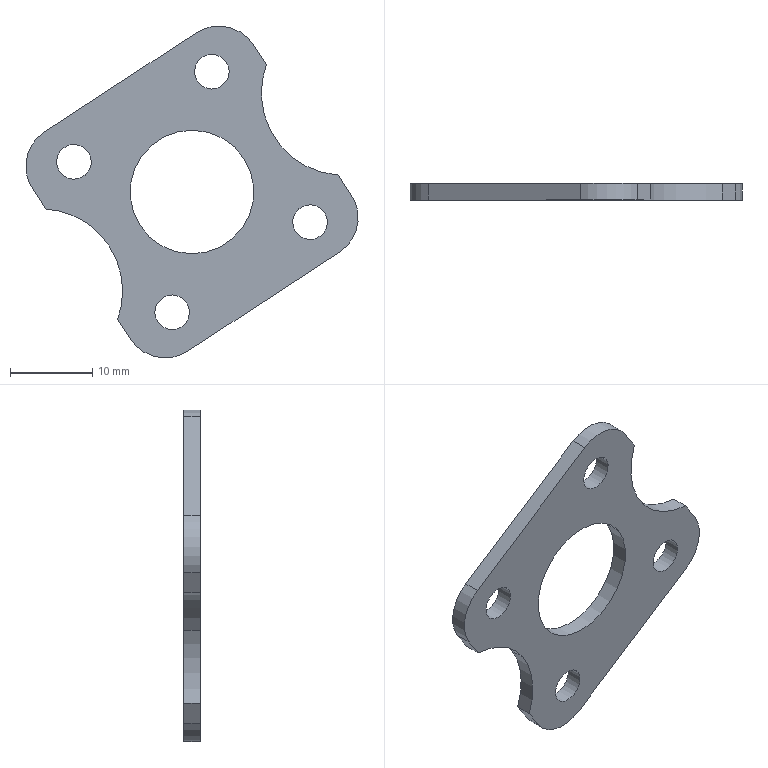Component | SolidWorks | FrontWheelPadPlate-2 | 1 solid | 25 faces | box 40.34 x 2 x 40.28 mm | volume 1349 mm3 | cylinder 17 | plane 8 | commonest cylinder face diameters 4.2 x8 10 x4 20 x3 15 x2
build123d program:
from build123d import *

# Parameters (mm, degrees)
SKETCH1_W           = 32
SKETCH1_H           = 31.8
SKETCH1_R           = 2.1
SKETCH1_R_2         = 7.5
BOSS_EXTRUDE1_DEPTH = 2
SKETCH2_R           = 10
CUT_EXTRUDE1_DEPTH  = 23.645
FILLET1_R           = 5


with BuildPart() as part:
    # Sketch1 → Boss-Extrude1 (new body)
    with BuildSketch(Plane.XY):
        Rectangle(SKETCH1_W, SKETCH1_H)
        with Locations((-10, 10.9)):
            Circle(SKETCH1_R, mode=Mode.SUBTRACT)
        with Locations(Location((10, 10.9, 0), (0, 0, 180))):
            Circle(SKETCH1_R, mode=Mode.SUBTRACT)
        with Locations((10, -10.9)):
            Circle(SKETCH1_R, mode=Mode.SUBTRACT)
        with Locations(Location((-10, -10.9, 0), (0, 0, 180))):
            Circle(SKETCH1_R, mode=Mode.SUBTRACT)
        Circle(SKETCH1_R_2, mode=Mode.SUBTRACT)
    extrude(amount=BOSS_EXTRUDE1_DEPTH)

    # Sketch2 → Cut-Extrude1 (cut, through all)
    with BuildSketch(Plane.XY.offset(2)):
        with Locations((22, 0)):
            Circle(SKETCH2_R)
        with Locations((-22, 0)):
            Circle(SKETCH2_R)
    extrude(amount=-CUT_EXTRUDE1_DEPTH, mode=Mode.SUBTRACT)

    # Fillet1
    fillet1_edges = [part.edges().sort_by_distance(p)[0] for p in [
        (16, -15.9, 1),
        (-16, -15.9, 1),
        (-16, 15.9, 1),
        (16, 15.9, 1),
    ]]
    fillet(fillet1_edges, radius=FILLET1_R)


solid = part.part

# Placed as in the assembly
solid = solid.moved(Location((0.3183, -13.6, 37), (90, 0, 33.158)))
STEP:
#1=CARTESIAN_POINT('',(-0.383,-0.6142,1.198));
#2=VERTEX_POINT('',#1);
#3=CARTESIAN_POINT('',(-0.3426,-0.6142,0.8485));
#4=VERTEX_POINT('',#3);
#5=CARTESIAN_POINT('',(-0.7126,-0.6142,0.983));
#6=DIRECTION('',(0.,1.,0.));
#7=DIRECTION('',(-0.8372,0.,-0.5469));
#8=AXIS2_PLACEMENT_3D('',#5,#6,#7);
#9=CIRCLE('',#8,0.3937);
#10=EDGE_CURVE('',#2,#4,#9,.T.);
#11=ORIENTED_EDGE('',*,*,#10,.F.);
#12=CARTESIAN_POINT('',(-0.383,-0.5354,1.198));
#13=VERTEX_POINT('',#12);
#14=CARTESIAN_POINT('',(-0.383,-0.6142,1.198));
#15=DIRECTION('',(0.,1.,0.));
#16=VECTOR('',#15,39.37);
#17=LINE('',#14,#16);
#18=EDGE_CURVE('',#2,#13,#17,.T.);
#19=ORIENTED_EDGE('',*,*,#18,.T.);
#20=CARTESIAN_POINT('',(-0.3426,-0.5354,0.8485));
#21=VERTEX_POINT('',#20);
#22=CARTESIAN_POINT('',(-0.7126,-0.5354,0.983));
#23=DIRECTION('',(0.,1.,0.));
#24=DIRECTION('',(-0.8372,0.,-0.5469));
#25=AXIS2_PLACEMENT_3D('',#22,#23,#24);
#26=CIRCLE('',#25,0.3937);
#27=EDGE_CURVE('',#13,#21,#26,.T.);
#28=ORIENTED_EDGE('',*,*,#27,.T.);
#29=CARTESIAN_POINT('',(-0.3426,-0.6142,0.8485));
#30=DIRECTION('',(0.,1.,0.));
#31=VECTOR('',#30,39.37);
#32=LINE('',#29,#31);
#33=EDGE_CURVE('',#4,#21,#32,.T.);
#34=ORIENTED_EDGE('',*,*,#33,.F.);
#35=EDGE_LOOP('',(#11,#19,#28,#34));
#36=FACE_OUTER_BOUND('',#35,.T.);
#37=CARTESIAN_POINT('',(-0.7126,-0.6142,0.983));
#38=DIRECTION('',(0.,1.,0.));
#39=DIRECTION('',(0.8372,0.,0.5469));
#40=AXIS2_PLACEMENT_3D('',#37,#38,#39);
#41=CYLINDRICAL_SURFACE('',#40,0.3937);
#42=ADVANCED_FACE('',(#36),#41,.F.);
#43=CARTESIAN_POINT('',(-0.2347,-0.5354,1.295));
#44=VERTEX_POINT('',#43);
#45=CARTESIAN_POINT('',(0.2597,-0.5354,1.618));
#46=VERTEX_POINT('',#45);
#47=CARTESIAN_POINT('',(0.01253,-0.5354,1.457));
#48=DIRECTION('',(0.,1.,0.));
#49=DIRECTION('',(0.8372,0.,0.5469));
#50=AXIS2_PLACEMENT_3D('',#47,#48,#49);
#51=CIRCLE('',#50,0.2953);
#52=EDGE_CURVE('',#44,#46,#51,.T.);
#53=ORIENTED_EDGE('',*,*,#52,.T.);
#54=CARTESIAN_POINT('',(0.2597,-0.6142,1.618));
#55=VERTEX_POINT('',#54);
#56=CARTESIAN_POINT('',(0.2597,-0.5354,1.618));
#57=DIRECTION('',(0.,-1.,0.));
#58=VECTOR('',#57,39.37);
#59=LINE('',#56,#58);
#60=EDGE_CURVE('',#46,#55,#59,.T.);
#61=ORIENTED_EDGE('',*,*,#60,.T.);
#62=CARTESIAN_POINT('',(-0.2347,-0.6142,1.295));
#63=VERTEX_POINT('',#62);
#64=CARTESIAN_POINT('',(0.01253,-0.6142,1.457));
#65=DIRECTION('',(0.,1.,0.));
#66=DIRECTION('',(0.8372,0.,0.5469));
#67=AXIS2_PLACEMENT_3D('',#64,#65,#66);
#68=CIRCLE('',#67,0.2953);
#69=EDGE_CURVE('',#63,#55,#68,.T.);
#70=ORIENTED_EDGE('',*,*,#69,.F.);
#71=CARTESIAN_POINT('',(-0.2347,-0.5354,1.295));
#72=DIRECTION('',(0.,-1.,0.));
#73=VECTOR('',#72,39.37);
#74=LINE('',#71,#73);
#75=EDGE_CURVE('',#44,#63,#74,.T.);
#76=ORIENTED_EDGE('',*,*,#75,.F.);
#77=EDGE_LOOP('',(#53,#61,#70,#76));
#78=FACE_OUTER_BOUND('',#77,.T.);
#79=CARTESIAN_POINT('',(0.01253,-0.5354,1.457));
#80=DIRECTION('',(0.,-1.,0.));
#81=DIRECTION('',(-0.8372,0.,-0.5469));
#82=AXIS2_PLACEMENT_3D('',#79,#80,#81);
#83=CYLINDRICAL_SURFACE('',#82,0.2953);
#84=ADVANCED_FACE('',(#78),#83,.F.);
#85=CARTESIAN_POINT('',(-0.621,-0.5354,1.555));
#86=VERTEX_POINT('',#85);
#87=CARTESIAN_POINT('',(-0.4826,-0.5354,1.646));
#88=VERTEX_POINT('',#87);
#89=CARTESIAN_POINT('',(-0.5518,-0.5354,1.601));
#90=DIRECTION('',(0.,1.,0.));
#91=DIRECTION('',(-0.8372,0.,-0.5469));
#92=AXIS2_PLACEMENT_3D('',#89,#90,#91);
#93=CIRCLE('',#92,0.08268);
#94=EDGE_CURVE('',#86,#88,#93,.T.);
#95=ORIENTED_EDGE('',*,*,#94,.T.);
#96=CARTESIAN_POINT('',(-0.4826,-0.6142,1.646));
#97=VERTEX_POINT('',#96);
#98=CARTESIAN_POINT('',(-0.4826,-0.5354,1.646));
#99=DIRECTION('',(0.,-1.,0.));
#100=VECTOR('',#99,39.37);
#101=LINE('',#98,#100);
#102=EDGE_CURVE('',#88,#97,#101,.T.);
#103=ORIENTED_EDGE('',*,*,#102,.T.);
#104=CARTESIAN_POINT('',(-0.621,-0.6142,1.555));
#105=VERTEX_POINT('',#104);
#106=CARTESIAN_POINT('',(-0.5518,-0.6142,1.601));
#107=DIRECTION('',(0.,1.,0.));
#108=DIRECTION('',(-0.8372,0.,-0.5469));
#109=AXIS2_PLACEMENT_3D('',#106,#107,#108);
#110=CIRCLE('',#109,0.08268);
#111=EDGE_CURVE('',#105,#97,#110,.T.);
#112=ORIENTED_EDGE('',*,*,#111,.F.);
#113=CARTESIAN_POINT('',(-0.621,-0.5354,1.555));
#114=DIRECTION('',(0.,-1.,0.));
#115=VECTOR('',#114,39.37);
#116=LINE('',#113,#115);
#117=EDGE_CURVE('',#86,#105,#116,.T.);
#118=ORIENTED_EDGE('',*,*,#117,.F.);
#119=EDGE_LOOP('',(#95,#103,#112,#118));
#120=FACE_OUTER_BOUND('',#119,.T.);
#121=CARTESIAN_POINT('',(-0.5518,-0.5354,1.601));
#122=DIRECTION('',(0.,-1.,0.));
#123=DIRECTION('',(-0.8372,0.,-0.5469));
#124=AXIS2_PLACEMENT_3D('',#121,#122,#123);
#125=CYLINDRICAL_SURFACE('',#124,0.08268);
#126=ADVANCED_FACE('',(#120),#125,.F.);
#127=CARTESIAN_POINT('',(0.0382,-0.5354,1.986));
#128=VERTEX_POINT('',#127);
#129=CARTESIAN_POINT('',(0.1766,-0.5354,2.077));
#130=VERTEX_POINT('',#129);
#131=CARTESIAN_POINT('',(0.1074,-0.5354,2.031));
#132=DIRECTION('',(0.,1.,0.));
#133=DIRECTION('',(0.8372,0.,0.5469));
#134=AXIS2_PLACEMENT_3D('',#131,#132,#133);
#135=CIRCLE('',#134,0.08268);
#136=EDGE_CURVE('',#128,#130,#135,.T.);
#137=ORIENTED_EDGE('',*,*,#136,.T.);
#138=CARTESIAN_POINT('',(0.1766,-0.6142,2.077));
#139=VERTEX_POINT('',#138);
#140=CARTESIAN_POINT('',(0.1766,-0.5354,2.077));
#141=DIRECTION('',(0.,-1.,0.));
#142=VECTOR('',#141,39.37);
#143=LINE('',#140,#142);
#144=EDGE_CURVE('',#130,#139,#143,.T.);
#145=ORIENTED_EDGE('',*,*,#144,.T.);
#146=CARTESIAN_POINT('',(0.0382,-0.6142,1.986));
#147=VERTEX_POINT('',#146);
#148=CARTESIAN_POINT('',(0.1074,-0.6142,2.031));
#149=DIRECTION('',(0.,1.,0.));
#150=DIRECTION('',(0.8372,0.,0.5469));
#151=AXIS2_PLACEMENT_3D('',#148,#149,#150);
#152=CIRCLE('',#151,0.08268);
#153=EDGE_CURVE('',#147,#139,#152,.T.);
#154=ORIENTED_EDGE('',*,*,#153,.F.);
#155=CARTESIAN_POINT('',(0.0382,-0.5354,1.986));
#156=DIRECTION('',(0.,-1.,0.));
#157=VECTOR('',#156,39.37);
#158=LINE('',#155,#157);
#159=EDGE_CURVE('',#128,#147,#158,.T.);
#160=ORIENTED_EDGE('',*,*,#159,.F.);
#161=EDGE_LOOP('',(#137,#145,#154,#160));
#162=FACE_OUTER_BOUND('',#161,.T.);
#163=CARTESIAN_POINT('',(0.1074,-0.5354,2.031));
#164=DIRECTION('',(0.,-1.,0.));
#165=DIRECTION('',(-0.8372,0.,-0.5469));
#166=AXIS2_PLACEMENT_3D('',#163,#164,#165);
#167=CYLINDRICAL_SURFACE('',#166,0.08268);
#168=ADVANCED_FACE('',(#162),#167,.F.);
#169=CARTESIAN_POINT('',(0.5076,-0.5354,1.268));
#170=VERTEX_POINT('',#169);
#171=CARTESIAN_POINT('',(0.6461,-0.5354,1.358));
#172=VERTEX_POINT('',#171);
#173=CARTESIAN_POINT('',(0.5768,-0.5354,1.313));
#174=DIRECTION('',(0.,1.,0.));
#175=DIRECTION('',(-0.8372,0.,-0.5469));
#176=AXIS2_PLACEMENT_3D('',#173,#174,#175);
#177=CIRCLE('',#176,0.08268);
#178=EDGE_CURVE('',#170,#172,#177,.T.);
#179=ORIENTED_EDGE('',*,*,#178,.T.);
#180=CARTESIAN_POINT('',(0.6461,-0.6142,1.358));
#181=VERTEX_POINT('',#180);
#182=CARTESIAN_POINT('',(0.6461,-0.5354,1.358));
#183=DIRECTION('',(0.,-1.,0.));
#184=VECTOR('',#183,39.37);
#185=LINE('',#182,#184);
#186=EDGE_CURVE('',#172,#181,#185,.T.);
#187=ORIENTED_EDGE('',*,*,#186,.T.);
#188=CARTESIAN_POINT('',(0.5076,-0.6142,1.268));
#189=VERTEX_POINT('',#188);
#190=CARTESIAN_POINT('',(0.5768,-0.6142,1.313));
#191=DIRECTION('',(0.,1.,0.));
#192=DIRECTION('',(-0.8372,0.,-0.5469));
#193=AXIS2_PLACEMENT_3D('',#190,#191,#192);
#194=CIRCLE('',#193,0.08268);
#195=EDGE_CURVE('',#189,#181,#194,.T.);
#196=ORIENTED_EDGE('',*,*,#195,.F.);
#197=CARTESIAN_POINT('',(0.5076,-0.5354,1.268));
#198=DIRECTION('',(0.,-1.,0.));
#199=VECTOR('',#198,39.37);
#200=LINE('',#197,#199);
#201=EDGE_CURVE('',#170,#189,#200,.T.);
#202=ORIENTED_EDGE('',*,*,#201,.F.);
#203=EDGE_LOOP('',(#179,#187,#196,#202));
#204=FACE_OUTER_BOUND('',#203,.T.);
#205=CARTESIAN_POINT('',(0.5768,-0.5354,1.313));
#206=DIRECTION('',(0.,-1.,0.));
#207=DIRECTION('',(-0.8372,0.,-0.5469));
#208=AXIS2_PLACEMENT_3D('',#205,#206,#207);
#209=CYLINDRICAL_SURFACE('',#208,0.08268);
#210=ADVANCED_FACE('',(#204),#209,.F.);
#211=CARTESIAN_POINT('',(-0.1516,-0.5354,0.8369));
#212=VERTEX_POINT('',#211);
#213=CARTESIAN_POINT('',(-0.01313,-0.5354,0.9273));
#214=VERTEX_POINT('',#213);
#215=CARTESIAN_POINT('',(-0.08235,-0.5354,0.8821));
#216=DIRECTION('',(0.,1.,0.));
#217=DIRECTION('',(0.8372,0.,0.5469));
#218=AXIS2_PLACEMENT_3D('',#215,#216,#217);
#219=CIRCLE('',#218,0.08268);
#220=EDGE_CURVE('',#212,#214,#219,.T.);
#221=ORIENTED_EDGE('',*,*,#220,.T.);
#222=CARTESIAN_POINT('',(-0.01313,-0.6142,0.9273));
#223=VERTEX_POINT('',#222);
#224=CARTESIAN_POINT('',(-0.01313,-0.5354,0.9273));
#225=DIRECTION('',(0.,-1.,0.));
#226=VECTOR('',#225,39.37);
#227=LINE('',#224,#226);
#228=EDGE_CURVE('',#214,#223,#227,.T.);
#229=ORIENTED_EDGE('',*,*,#228,.T.);
#230=CARTESIAN_POINT('',(-0.1516,-0.6142,0.8369));
#231=VERTEX_POINT('',#230);
#232=CARTESIAN_POINT('',(-0.08235,-0.6142,0.8821));
#233=DIRECTION('',(0.,1.,0.));
#234=DIRECTION('',(0.8372,0.,0.5469));
#235=AXIS2_PLACEMENT_3D('',#232,#233,#234);
#236=CIRCLE('',#235,0.08268);
#237=EDGE_CURVE('',#231,#223,#236,.T.);
#238=ORIENTED_EDGE('',*,*,#237,.F.);
#239=CARTESIAN_POINT('',(-0.1516,-0.5354,0.8369));
#240=DIRECTION('',(0.,-1.,0.));
#241=VECTOR('',#240,39.37);
#242=LINE('',#239,#241);
#243=EDGE_CURVE('',#212,#231,#242,.T.);
#244=ORIENTED_EDGE('',*,*,#243,.F.);
#245=EDGE_LOOP('',(#221,#229,#238,#244));
#246=FACE_OUTER_BOUND('',#245,.T.);
#247=CARTESIAN_POINT('',(-0.08235,-0.5354,0.8821));
#248=DIRECTION('',(0.,-1.,0.));
#249=DIRECTION('',(-0.8372,0.,-0.5469));
#250=AXIS2_PLACEMENT_3D('',#247,#248,#249);
#251=CYLINDRICAL_SURFACE('',#250,0.08268);
#252=ADVANCED_FACE('',(#246),#251,.F.);
#253=CARTESIAN_POINT('',(-0.2801,-0.5354,0.7529));
#254=VERTEX_POINT('',#253);
#255=CARTESIAN_POINT('',(-0.8572,-0.5354,1.636));
#256=DIRECTION('',(-0.5469,0.,0.8372));
#257=VECTOR('',#256,39.37);
#258=LINE('',#255,#257);
#259=EDGE_CURVE('',#254,#21,#258,.T.);
#260=ORIENTED_EDGE('',*,*,#259,.F.);
#261=CARTESIAN_POINT('',(-0.2801,-0.6142,0.7529));
#262=VERTEX_POINT('',#261);
#263=CARTESIAN_POINT('',(-0.2801,-0.5354,0.7529));
#264=DIRECTION('',(0.,-1.,0.));
#265=VECTOR('',#264,39.37);
#266=LINE('',#263,#265);
#267=EDGE_CURVE('',#254,#262,#266,.T.);
#268=ORIENTED_EDGE('',*,*,#267,.T.);
#269=CARTESIAN_POINT('',(-0.8572,-0.6142,1.636));
#270=DIRECTION('',(-0.5469,0.,0.8372));
#271=VECTOR('',#270,39.37);
#272=LINE('',#269,#271);
#273=EDGE_CURVE('',#262,#4,#272,.T.);
#274=ORIENTED_EDGE('',*,*,#273,.T.);
#275=ORIENTED_EDGE('',*,*,#33,.T.);
#276=EDGE_LOOP('',(#260,#268,#274,#275));
#277=FACE_OUTER_BOUND('',#276,.T.);
#278=CARTESIAN_POINT('',(-0.8572,-0.5354,1.636));
#279=DIRECTION('',(0.8372,0.,0.5469));
#280=DIRECTION('',(0.,-1.,0.));
#281=AXIS2_PLACEMENT_3D('',#278,#279,#280);
#282=PLANE('',#281);
#283=ADVANCED_FACE('',(#277),#282,.F.);
#284=CARTESIAN_POINT('',(0.3052,-0.5354,2.16));
#285=VERTEX_POINT('',#284);
#286=CARTESIAN_POINT('',(0.3676,-0.5354,2.065));
#287=VERTEX_POINT('',#286);
#288=CARTESIAN_POINT('',(0.1975,-0.5354,2.325));
#289=DIRECTION('',(0.5469,0.,-0.8372));
#290=VECTOR('',#289,39.37);
#291=LINE('',#288,#290);
#292=EDGE_CURVE('',#285,#287,#291,.T.);
#293=ORIENTED_EDGE('',*,*,#292,.F.);
#294=CARTESIAN_POINT('',(0.3052,-0.6142,2.16));
#295=VERTEX_POINT('',#294);
#296=CARTESIAN_POINT('',(0.3052,-0.5354,2.16));
#297=DIRECTION('',(0.,-1.,0.));
#298=VECTOR('',#297,39.37);
#299=LINE('',#296,#298);
#300=EDGE_CURVE('',#285,#295,#299,.T.);
#301=ORIENTED_EDGE('',*,*,#300,.T.);
#302=CARTESIAN_POINT('',(0.3676,-0.6142,2.065));
#303=VERTEX_POINT('',#302);
#304=CARTESIAN_POINT('',(0.1975,-0.6142,2.325));
#305=DIRECTION('',(0.5469,0.,-0.8372));
#306=VECTOR('',#305,39.37);
#307=LINE('',#304,#306);
#308=EDGE_CURVE('',#295,#303,#307,.T.);
#309=ORIENTED_EDGE('',*,*,#308,.T.);
#310=CARTESIAN_POINT('',(0.3676,-0.6142,2.065));
#311=DIRECTION('',(0.,1.,0.));
#312=VECTOR('',#311,39.37);
#313=LINE('',#310,#312);
#314=EDGE_CURVE('',#303,#287,#313,.T.);
#315=ORIENTED_EDGE('',*,*,#314,.T.);
#316=EDGE_LOOP('',(#293,#301,#309,#315));
#317=FACE_OUTER_BOUND('',#316,.T.);
#318=CARTESIAN_POINT('',(0.1975,-0.5354,2.325));
#319=DIRECTION('',(-0.8372,0.,-0.5469));
#320=DIRECTION('',(0.,1.,0.));
#321=AXIS2_PLACEMENT_3D('',#318,#319,#320);
#322=PLANE('',#321);
#323=ADVANCED_FACE('',(#317),#322,.F.);
#324=CARTESIAN_POINT('',(-0.6871,-0.5354,1.376));
#325=VERTEX_POINT('',#324);
#326=CARTESIAN_POINT('',(-0.7495,-0.5354,1.471));
#327=VERTEX_POINT('',#326);
#328=CARTESIAN_POINT('',(-0.8572,-0.5354,1.636));
#329=DIRECTION('',(-0.5469,0.,0.8372));
#330=VECTOR('',#329,39.37);
#331=LINE('',#328,#330);
#332=EDGE_CURVE('',#325,#327,#331,.T.);
#333=ORIENTED_EDGE('',*,*,#332,.T.);
#334=CARTESIAN_POINT('',(-0.6924,-0.5354,1.744));
#335=VERTEX_POINT('',#334);
#336=CARTESIAN_POINT('',(-0.5847,-0.5354,1.579));
#337=DIRECTION('',(0.,1.,0.));
#338=DIRECTION('',(-0.8372,0.,-0.5469));
#339=AXIS2_PLACEMENT_3D('',#336,#337,#338);
#340=CIRCLE('',#339,0.1969);
#341=EDGE_CURVE('',#327,#335,#340,.T.);
#342=ORIENTED_EDGE('',*,*,#341,.T.);
#343=CARTESIAN_POINT('',(0.03271,-0.5354,2.218));
#344=VERTEX_POINT('',#343);
#345=CARTESIAN_POINT('',(-0.8572,-0.5354,1.636));
#346=DIRECTION('',(0.8372,0.,0.5469));
#347=VECTOR('',#346,39.37);
#348=LINE('',#345,#347);
#349=EDGE_CURVE('',#335,#344,#348,.T.);
#350=ORIENTED_EDGE('',*,*,#349,.T.);
#351=CARTESIAN_POINT('',(0.1404,-0.5354,2.053));
#352=DIRECTION('',(0.,1.,0.));
#353=DIRECTION('',(-0.8372,0.,-0.5469));
#354=AXIS2_PLACEMENT_3D('',#351,#352,#353);
#355=CIRCLE('',#354,0.1969);
#356=EDGE_CURVE('',#344,#285,#355,.T.);
#357=ORIENTED_EDGE('',*,*,#356,.T.);
#358=ORIENTED_EDGE('',*,*,#292,.T.);
#359=CARTESIAN_POINT('',(0.7121,-0.5354,1.538));
#360=VERTEX_POINT('',#359);
#361=CARTESIAN_POINT('',(0.7376,-0.5354,1.93));
#362=DIRECTION('',(0.,1.,0.));
#363=DIRECTION('',(0.8372,0.,0.5469));
#364=AXIS2_PLACEMENT_3D('',#361,#362,#363);
#365=CIRCLE('',#364,0.3937);
#366=EDGE_CURVE('',#360,#287,#365,.T.);
#367=ORIENTED_EDGE('',*,*,#366,.F.);
#368=CARTESIAN_POINT('',(0.7746,-0.5354,1.442));
#369=VERTEX_POINT('',#368);
#370=CARTESIAN_POINT('',(0.1975,-0.5354,2.325));
#371=DIRECTION('',(0.5469,0.,-0.8372));
#372=VECTOR('',#371,39.37);
#373=LINE('',#370,#372);
#374=EDGE_CURVE('',#360,#369,#373,.T.);
#375=ORIENTED_EDGE('',*,*,#374,.T.);
#376=CARTESIAN_POINT('',(0.7175,-0.5354,1.17));
#377=VERTEX_POINT('',#376);
#378=CARTESIAN_POINT('',(0.6098,-0.5354,1.334));
#379=DIRECTION('',(0.,1.,0.));
#380=DIRECTION('',(-0.8372,0.,-0.5469));
#381=AXIS2_PLACEMENT_3D('',#378,#379,#380);
#382=CIRCLE('',#381,0.1969);
#383=EDGE_CURVE('',#369,#377,#382,.T.);
#384=ORIENTED_EDGE('',*,*,#383,.T.);
#385=CARTESIAN_POINT('',(-0.007642,-0.5354,0.6958));
#386=VERTEX_POINT('',#385);
#387=CARTESIAN_POINT('',(-0.1724,-0.5354,0.5881));
#388=DIRECTION('',(-0.8372,0.,-0.5469));
#389=VECTOR('',#388,39.37);
#390=LINE('',#387,#389);
#391=EDGE_CURVE('',#377,#386,#390,.T.);
#392=ORIENTED_EDGE('',*,*,#391,.T.);
#393=CARTESIAN_POINT('',(-0.1153,-0.5354,0.8606));
#394=DIRECTION('',(0.,1.,0.));
#395=DIRECTION('',(-0.8372,0.,-0.5469));
#396=AXIS2_PLACEMENT_3D('',#393,#394,#395);
#397=CIRCLE('',#396,0.1969);
#398=EDGE_CURVE('',#386,#254,#397,.T.);
#399=ORIENTED_EDGE('',*,*,#398,.T.);
#400=ORIENTED_EDGE('',*,*,#259,.T.);
#401=ORIENTED_EDGE('',*,*,#27,.F.);
#402=CARTESIAN_POINT('',(-0.7126,-0.5354,0.983));
#403=DIRECTION('',(0.,1.,0.));
#404=DIRECTION('',(-0.8372,0.,-0.5469));
#405=AXIS2_PLACEMENT_3D('',#402,#403,#404);
#406=CIRCLE('',#405,0.3937);
#407=EDGE_CURVE('',#325,#13,#406,.T.);
#408=ORIENTED_EDGE('',*,*,#407,.F.);
#409=EDGE_LOOP('',(#333,#342,#350,#357,#358,#367,#375,#384,#392,#399,#400,#401,#408));
#410=FACE_OUTER_BOUND('',#409,.T.);
#411=ORIENTED_EDGE('',*,*,#220,.F.);
#412=CARTESIAN_POINT('',(-0.08235,-0.5354,0.8821));
#413=DIRECTION('',(0.,1.,0.));
#414=DIRECTION('',(0.8372,0.,0.5469));
#415=AXIS2_PLACEMENT_3D('',#412,#413,#414);
#416=CIRCLE('',#415,0.08268);
#417=EDGE_CURVE('',#214,#212,#416,.T.);
#418=ORIENTED_EDGE('',*,*,#417,.F.);
#419=EDGE_LOOP('',(#411,#418));
#420=FACE_BOUND('',#419,.T.);
#421=ORIENTED_EDGE('',*,*,#178,.F.);
#422=CARTESIAN_POINT('',(0.5768,-0.5354,1.313));
#423=DIRECTION('',(0.,1.,0.));
#424=DIRECTION('',(-0.8372,0.,-0.5469));
#425=AXIS2_PLACEMENT_3D('',#422,#423,#424);
#426=CIRCLE('',#425,0.08268);
#427=EDGE_CURVE('',#172,#170,#426,.T.);
#428=ORIENTED_EDGE('',*,*,#427,.F.);
#429=EDGE_LOOP('',(#421,#428));
#430=FACE_BOUND('',#429,.T.);
#431=ORIENTED_EDGE('',*,*,#136,.F.);
#432=CARTESIAN_POINT('',(0.1074,-0.5354,2.031));
#433=DIRECTION('',(0.,1.,0.));
#434=DIRECTION('',(0.8372,0.,0.5469));
#435=AXIS2_PLACEMENT_3D('',#432,#433,#434);
#436=CIRCLE('',#435,0.08268);
#437=EDGE_CURVE('',#130,#128,#436,.T.);
#438=ORIENTED_EDGE('',*,*,#437,.F.);
#439=EDGE_LOOP('',(#431,#438));
#440=FACE_BOUND('',#439,.T.);
#441=ORIENTED_EDGE('',*,*,#94,.F.);
#442=CARTESIAN_POINT('',(-0.5518,-0.5354,1.601));
#443=DIRECTION('',(0.,1.,0.));
#444=DIRECTION('',(-0.8372,0.,-0.5469));
#445=AXIS2_PLACEMENT_3D('',#442,#443,#444);
#446=CIRCLE('',#445,0.08268);
#447=EDGE_CURVE('',#88,#86,#446,.T.);
#448=ORIENTED_EDGE('',*,*,#447,.F.);
#449=EDGE_LOOP('',(#441,#448));
#450=FACE_BOUND('',#449,.T.);
#451=ORIENTED_EDGE('',*,*,#52,.F.);
#452=CARTESIAN_POINT('',(0.01253,-0.5354,1.457));
#453=DIRECTION('',(0.,1.,0.));
#454=DIRECTION('',(0.8372,0.,0.5469));
#455=AXIS2_PLACEMENT_3D('',#452,#453,#454);
#456=CIRCLE('',#455,0.2953);
#457=EDGE_CURVE('',#46,#44,#456,.T.);
#458=ORIENTED_EDGE('',*,*,#457,.F.);
#459=EDGE_LOOP('',(#451,#458));
#460=FACE_BOUND('',#459,.T.);
#461=CARTESIAN_POINT('',(0.01253,-0.5354,1.457));
#462=DIRECTION('',(0.,-1.,0.));
#463=DIRECTION('',(-0.8372,0.,-0.5469));
#464=AXIS2_PLACEMENT_3D('',#461,#462,#463);
#465=PLANE('',#464);
#466=ADVANCED_FACE('',(#410,#420,#430,#440,#450,#460),#465,.F.);
#467=CARTESIAN_POINT('',(-0.6924,-0.6142,1.744));
#468=VERTEX_POINT('',#467);
#469=CARTESIAN_POINT('',(0.03271,-0.6142,2.218));
#470=VERTEX_POINT('',#469);
#471=CARTESIAN_POINT('',(-0.8572,-0.6142,1.636));
#472=DIRECTION('',(0.8372,0.,0.5469));
#473=VECTOR('',#472,39.37);
#474=LINE('',#471,#473);
#475=EDGE_CURVE('',#468,#470,#474,.T.);
#476=ORIENTED_EDGE('',*,*,#475,.F.);
#477=CARTESIAN_POINT('',(-0.7495,-0.6142,1.471));
#478=VERTEX_POINT('',#477);
#479=CARTESIAN_POINT('',(-0.5847,-0.6142,1.579));
#480=DIRECTION('',(0.,-1.,0.));
#481=DIRECTION('',(-0.8372,0.,-0.5469));
#482=AXIS2_PLACEMENT_3D('',#479,#480,#481);
#483=CIRCLE('',#482,0.1969);
#484=EDGE_CURVE('',#468,#478,#483,.T.);
#485=ORIENTED_EDGE('',*,*,#484,.T.);
#486=CARTESIAN_POINT('',(-0.6871,-0.6142,1.376));
#487=VERTEX_POINT('',#486);
#488=CARTESIAN_POINT('',(-0.8572,-0.6142,1.636));
#489=DIRECTION('',(-0.5469,0.,0.8372));
#490=VECTOR('',#489,39.37);
#491=LINE('',#488,#490);
#492=EDGE_CURVE('',#487,#478,#491,.T.);
#493=ORIENTED_EDGE('',*,*,#492,.F.);
#494=CARTESIAN_POINT('',(-0.7126,-0.6142,0.983));
#495=DIRECTION('',(0.,1.,0.));
#496=DIRECTION('',(-0.8372,0.,-0.5469));
#497=AXIS2_PLACEMENT_3D('',#494,#495,#496);
#498=CIRCLE('',#497,0.3937);
#499=EDGE_CURVE('',#487,#2,#498,.T.);
#500=ORIENTED_EDGE('',*,*,#499,.T.);
#501=ORIENTED_EDGE('',*,*,#10,.T.);
#502=ORIENTED_EDGE('',*,*,#273,.F.);
#503=CARTESIAN_POINT('',(-0.007642,-0.6142,0.6958));
#504=VERTEX_POINT('',#503);
#505=CARTESIAN_POINT('',(-0.1153,-0.6142,0.8606));
#506=DIRECTION('',(0.,-1.,0.));
#507=DIRECTION('',(-0.8372,0.,-0.5469));
#508=AXIS2_PLACEMENT_3D('',#505,#506,#507);
#509=CIRCLE('',#508,0.1969);
#510=EDGE_CURVE('',#262,#504,#509,.T.);
#511=ORIENTED_EDGE('',*,*,#510,.T.);
#512=CARTESIAN_POINT('',(0.7175,-0.6142,1.17));
#513=VERTEX_POINT('',#512);
#514=CARTESIAN_POINT('',(-0.1724,-0.6142,0.5881));
#515=DIRECTION('',(-0.8372,0.,-0.5469));
#516=VECTOR('',#515,39.37);
#517=LINE('',#514,#516);
#518=EDGE_CURVE('',#513,#504,#517,.T.);
#519=ORIENTED_EDGE('',*,*,#518,.F.);
#520=CARTESIAN_POINT('',(0.7746,-0.6142,1.442));
#521=VERTEX_POINT('',#520);
#522=CARTESIAN_POINT('',(0.6098,-0.6142,1.334));
#523=DIRECTION('',(0.,-1.,0.));
#524=DIRECTION('',(-0.8372,0.,-0.5469));
#525=AXIS2_PLACEMENT_3D('',#522,#523,#524);
#526=CIRCLE('',#525,0.1969);
#527=EDGE_CURVE('',#513,#521,#526,.T.);
#528=ORIENTED_EDGE('',*,*,#527,.T.);
#529=CARTESIAN_POINT('',(0.7121,-0.6142,1.538));
#530=VERTEX_POINT('',#529);
#531=CARTESIAN_POINT('',(0.1975,-0.6142,2.325));
#532=DIRECTION('',(0.5469,0.,-0.8372));
#533=VECTOR('',#532,39.37);
#534=LINE('',#531,#533);
#535=EDGE_CURVE('',#530,#521,#534,.T.);
#536=ORIENTED_EDGE('',*,*,#535,.F.);
#537=CARTESIAN_POINT('',(0.7376,-0.6142,1.93));
#538=DIRECTION('',(0.,1.,0.));
#539=DIRECTION('',(0.8372,0.,0.5469));
#540=AXIS2_PLACEMENT_3D('',#537,#538,#539);
#541=CIRCLE('',#540,0.3937);
#542=EDGE_CURVE('',#530,#303,#541,.T.);
#543=ORIENTED_EDGE('',*,*,#542,.T.);
#544=ORIENTED_EDGE('',*,*,#308,.F.);
#545=CARTESIAN_POINT('',(0.1404,-0.6142,2.053));
#546=DIRECTION('',(0.,-1.,0.));
#547=DIRECTION('',(-0.8372,0.,-0.5469));
#548=AXIS2_PLACEMENT_3D('',#545,#546,#547);
#549=CIRCLE('',#548,0.1969);
#550=EDGE_CURVE('',#295,#470,#549,.T.);
#551=ORIENTED_EDGE('',*,*,#550,.T.);
#552=EDGE_LOOP('',(#476,#485,#493,#500,#501,#502,#511,#519,#528,#536,#543,#544,#551));
#553=FACE_OUTER_BOUND('',#552,.T.);
#554=ORIENTED_EDGE('',*,*,#111,.T.);
#555=CARTESIAN_POINT('',(-0.5518,-0.6142,1.601));
#556=DIRECTION('',(0.,1.,0.));
#557=DIRECTION('',(-0.8372,0.,-0.5469));
#558=AXIS2_PLACEMENT_3D('',#555,#556,#557);
#559=CIRCLE('',#558,0.08268);
#560=EDGE_CURVE('',#97,#105,#559,.T.);
#561=ORIENTED_EDGE('',*,*,#560,.T.);
#562=EDGE_LOOP('',(#554,#561));
#563=FACE_BOUND('',#562,.T.);
#564=ORIENTED_EDGE('',*,*,#195,.T.);
#565=CARTESIAN_POINT('',(0.5768,-0.6142,1.313));
#566=DIRECTION('',(0.,1.,0.));
#567=DIRECTION('',(-0.8372,0.,-0.5469));
#568=AXIS2_PLACEMENT_3D('',#565,#566,#567);
#569=CIRCLE('',#568,0.08268);
#570=EDGE_CURVE('',#181,#189,#569,.T.);
#571=ORIENTED_EDGE('',*,*,#570,.T.);
#572=EDGE_LOOP('',(#564,#571));
#573=FACE_BOUND('',#572,.T.);
#574=ORIENTED_EDGE('',*,*,#237,.T.);
#575=CARTESIAN_POINT('',(-0.08235,-0.6142,0.8821));
#576=DIRECTION('',(0.,1.,0.));
#577=DIRECTION('',(0.8372,0.,0.5469));
#578=AXIS2_PLACEMENT_3D('',#575,#576,#577);
#579=CIRCLE('',#578,0.08268);
#580=EDGE_CURVE('',#223,#231,#579,.T.);
#581=ORIENTED_EDGE('',*,*,#580,.T.);
#582=EDGE_LOOP('',(#574,#581));
#583=FACE_BOUND('',#582,.T.);
#584=ORIENTED_EDGE('',*,*,#153,.T.);
#585=CARTESIAN_POINT('',(0.1074,-0.6142,2.031));
#586=DIRECTION('',(0.,1.,0.));
#587=DIRECTION('',(0.8372,0.,0.5469));
#588=AXIS2_PLACEMENT_3D('',#585,#586,#587);
#589=CIRCLE('',#588,0.08268);
#590=EDGE_CURVE('',#139,#147,#589,.T.);
#591=ORIENTED_EDGE('',*,*,#590,.T.);
#592=EDGE_LOOP('',(#584,#591));
#593=FACE_BOUND('',#592,.T.);
#594=ORIENTED_EDGE('',*,*,#69,.T.);
#595=CARTESIAN_POINT('',(0.01253,-0.6142,1.457));
#596=DIRECTION('',(0.,1.,0.));
#597=DIRECTION('',(0.8372,0.,0.5469));
#598=AXIS2_PLACEMENT_3D('',#595,#596,#597);
#599=CIRCLE('',#598,0.2953);
#600=EDGE_CURVE('',#55,#63,#599,.T.);
#601=ORIENTED_EDGE('',*,*,#600,.T.);
#602=EDGE_LOOP('',(#594,#601));
#603=FACE_BOUND('',#602,.T.);
#604=CARTESIAN_POINT('',(0.01253,-0.6142,1.457));
#605=DIRECTION('',(0.,-1.,0.));
#606=DIRECTION('',(-0.8372,0.,-0.5469));
#607=AXIS2_PLACEMENT_3D('',#604,#605,#606);
#608=PLANE('',#607);
#609=ADVANCED_FACE('',(#553,#563,#573,#583,#593,#603),#608,.T.);
#610=ORIENTED_EDGE('',*,*,#535,.T.);
#611=CARTESIAN_POINT('',(0.7746,-0.5354,1.442));
#612=DIRECTION('',(0.,1.,0.));
#613=VECTOR('',#612,39.37);
#614=LINE('',#611,#613);
#615=EDGE_CURVE('',#521,#369,#614,.T.);
#616=ORIENTED_EDGE('',*,*,#615,.T.);
#617=ORIENTED_EDGE('',*,*,#374,.F.);
#618=CARTESIAN_POINT('',(0.7121,-0.6142,1.538));
#619=DIRECTION('',(0.,-1.,0.));
#620=VECTOR('',#619,39.37);
#621=LINE('',#618,#620);
#622=EDGE_CURVE('',#360,#530,#621,.T.);
#623=ORIENTED_EDGE('',*,*,#622,.T.);
#624=EDGE_LOOP('',(#610,#616,#617,#623));
#625=FACE_OUTER_BOUND('',#624,.T.);
#626=CARTESIAN_POINT('',(0.1975,-0.5354,2.325));
#627=DIRECTION('',(-0.8372,0.,-0.5469));
#628=DIRECTION('',(0.,1.,0.));
#629=AXIS2_PLACEMENT_3D('',#626,#627,#628);
#630=PLANE('',#629);
#631=ADVANCED_FACE('',(#625),#630,.F.);
#632=ORIENTED_EDGE('',*,*,#391,.F.);
#633=CARTESIAN_POINT('',(0.7175,-0.5354,1.17));
#634=DIRECTION('',(0.,-1.,0.));
#635=VECTOR('',#634,39.37);
#636=LINE('',#633,#635);
#637=EDGE_CURVE('',#377,#513,#636,.T.);
#638=ORIENTED_EDGE('',*,*,#637,.T.);
#639=ORIENTED_EDGE('',*,*,#518,.T.);
#640=CARTESIAN_POINT('',(-0.007642,-0.5354,0.6958));
#641=DIRECTION('',(0.,1.,0.));
#642=VECTOR('',#641,39.37);
#643=LINE('',#640,#642);
#644=EDGE_CURVE('',#504,#386,#643,.T.);
#645=ORIENTED_EDGE('',*,*,#644,.T.);
#646=EDGE_LOOP('',(#632,#638,#639,#645));
#647=FACE_OUTER_BOUND('',#646,.T.);
#648=CARTESIAN_POINT('',(-0.1724,-0.5354,0.5881));
#649=DIRECTION('',(-0.5469,0.,0.8372));
#650=DIRECTION('',(0.,-1.,0.));
#651=AXIS2_PLACEMENT_3D('',#648,#649,#650);
#652=PLANE('',#651);
#653=ADVANCED_FACE('',(#647),#652,.F.);
#654=ORIENTED_EDGE('',*,*,#492,.T.);
#655=CARTESIAN_POINT('',(-0.7495,-0.5354,1.471));
#656=DIRECTION('',(0.,1.,0.));
#657=VECTOR('',#656,39.37);
#658=LINE('',#655,#657);
#659=EDGE_CURVE('',#478,#327,#658,.T.);
#660=ORIENTED_EDGE('',*,*,#659,.T.);
#661=ORIENTED_EDGE('',*,*,#332,.F.);
#662=CARTESIAN_POINT('',(-0.6871,-0.6142,1.376));
#663=DIRECTION('',(0.,-1.,0.));
#664=VECTOR('',#663,39.37);
#665=LINE('',#662,#664);
#666=EDGE_CURVE('',#325,#487,#665,.T.);
#667=ORIENTED_EDGE('',*,*,#666,.T.);
#668=EDGE_LOOP('',(#654,#660,#661,#667));
#669=FACE_OUTER_BOUND('',#668,.T.);
#670=CARTESIAN_POINT('',(-0.8572,-0.5354,1.636));
#671=DIRECTION('',(0.8372,0.,0.5469));
#672=DIRECTION('',(0.,-1.,0.));
#673=AXIS2_PLACEMENT_3D('',#670,#671,#672);
#674=PLANE('',#673);
#675=ADVANCED_FACE('',(#669),#674,.F.);
#676=ORIENTED_EDGE('',*,*,#349,.F.);
#677=CARTESIAN_POINT('',(-0.6924,-0.5354,1.744));
#678=DIRECTION('',(0.,-1.,0.));
#679=VECTOR('',#678,39.37);
#680=LINE('',#677,#679);
#681=EDGE_CURVE('',#335,#468,#680,.T.);
#682=ORIENTED_EDGE('',*,*,#681,.T.);
#683=ORIENTED_EDGE('',*,*,#475,.T.);
#684=CARTESIAN_POINT('',(0.03271,-0.5354,2.218));
#685=DIRECTION('',(0.,1.,0.));
#686=VECTOR('',#685,39.37);
#687=LINE('',#684,#686);
#688=EDGE_CURVE('',#470,#344,#687,.T.);
#689=ORIENTED_EDGE('',*,*,#688,.T.);
#690=EDGE_LOOP('',(#676,#682,#683,#689));
#691=FACE_OUTER_BOUND('',#690,.T.);
#692=CARTESIAN_POINT('',(-0.8572,-0.5354,1.636));
#693=DIRECTION('',(0.5469,0.,-0.8372));
#694=DIRECTION('',(0.,1.,0.));
#695=AXIS2_PLACEMENT_3D('',#692,#693,#694);
#696=PLANE('',#695);
#697=ADVANCED_FACE('',(#691),#696,.F.);
#698=ORIENTED_EDGE('',*,*,#228,.F.);
#699=ORIENTED_EDGE('',*,*,#417,.T.);
#700=ORIENTED_EDGE('',*,*,#243,.T.);
#701=ORIENTED_EDGE('',*,*,#580,.F.);
#702=EDGE_LOOP('',(#698,#699,#700,#701));
#703=FACE_OUTER_BOUND('',#702,.T.);
#704=CARTESIAN_POINT('',(-0.08235,-0.5354,0.8821));
#705=DIRECTION('',(0.,-1.,0.));
#706=DIRECTION('',(-0.8372,0.,-0.5469));
#707=AXIS2_PLACEMENT_3D('',#704,#705,#706);
#708=CYLINDRICAL_SURFACE('',#707,0.08268);
#709=ADVANCED_FACE('',(#703),#708,.F.);
#710=ORIENTED_EDGE('',*,*,#186,.F.);
#711=ORIENTED_EDGE('',*,*,#427,.T.);
#712=ORIENTED_EDGE('',*,*,#201,.T.);
#713=ORIENTED_EDGE('',*,*,#570,.F.);
#714=EDGE_LOOP('',(#710,#711,#712,#713));
#715=FACE_OUTER_BOUND('',#714,.T.);
#716=CARTESIAN_POINT('',(0.5768,-0.5354,1.313));
#717=DIRECTION('',(0.,-1.,0.));
#718=DIRECTION('',(-0.8372,0.,-0.5469));
#719=AXIS2_PLACEMENT_3D('',#716,#717,#718);
#720=CYLINDRICAL_SURFACE('',#719,0.08268);
#721=ADVANCED_FACE('',(#715),#720,.F.);
#722=ORIENTED_EDGE('',*,*,#144,.F.);
#723=ORIENTED_EDGE('',*,*,#437,.T.);
#724=ORIENTED_EDGE('',*,*,#159,.T.);
#725=ORIENTED_EDGE('',*,*,#590,.F.);
#726=EDGE_LOOP('',(#722,#723,#724,#725));
#727=FACE_OUTER_BOUND('',#726,.T.);
#728=CARTESIAN_POINT('',(0.1074,-0.5354,2.031));
#729=DIRECTION('',(0.,-1.,0.));
#730=DIRECTION('',(-0.8372,0.,-0.5469));
#731=AXIS2_PLACEMENT_3D('',#728,#729,#730);
#732=CYLINDRICAL_SURFACE('',#731,0.08268);
#733=ADVANCED_FACE('',(#727),#732,.F.);
#734=ORIENTED_EDGE('',*,*,#102,.F.);
#735=ORIENTED_EDGE('',*,*,#447,.T.);
#736=ORIENTED_EDGE('',*,*,#117,.T.);
#737=ORIENTED_EDGE('',*,*,#560,.F.);
#738=EDGE_LOOP('',(#734,#735,#736,#737));
#739=FACE_OUTER_BOUND('',#738,.T.);
#740=CARTESIAN_POINT('',(-0.5518,-0.5354,1.601));
#741=DIRECTION('',(0.,-1.,0.));
#742=DIRECTION('',(-0.8372,0.,-0.5469));
#743=AXIS2_PLACEMENT_3D('',#740,#741,#742);
#744=CYLINDRICAL_SURFACE('',#743,0.08268);
#745=ADVANCED_FACE('',(#739),#744,.F.);
#746=ORIENTED_EDGE('',*,*,#60,.F.);
#747=ORIENTED_EDGE('',*,*,#457,.T.);
#748=ORIENTED_EDGE('',*,*,#75,.T.);
#749=ORIENTED_EDGE('',*,*,#600,.F.);
#750=EDGE_LOOP('',(#746,#747,#748,#749));
#751=FACE_OUTER_BOUND('',#750,.T.);
#752=CARTESIAN_POINT('',(0.01253,-0.5354,1.457));
#753=DIRECTION('',(0.,-1.,0.));
#754=DIRECTION('',(-0.8372,0.,-0.5469));
#755=AXIS2_PLACEMENT_3D('',#752,#753,#754);
#756=CYLINDRICAL_SURFACE('',#755,0.2953);
#757=ADVANCED_FACE('',(#751),#756,.F.);
#758=ORIENTED_EDGE('',*,*,#542,.F.);
#759=ORIENTED_EDGE('',*,*,#622,.F.);
#760=ORIENTED_EDGE('',*,*,#366,.T.);
#761=ORIENTED_EDGE('',*,*,#314,.F.);
#762=EDGE_LOOP('',(#758,#759,#760,#761));
#763=FACE_OUTER_BOUND('',#762,.T.);
#764=CARTESIAN_POINT('',(0.7376,-0.6142,1.93));
#765=DIRECTION('',(0.,1.,0.));
#766=DIRECTION('',(0.8372,0.,0.5469));
#767=AXIS2_PLACEMENT_3D('',#764,#765,#766);
#768=CYLINDRICAL_SURFACE('',#767,0.3937);
#769=ADVANCED_FACE('',(#763),#768,.F.);
#770=ORIENTED_EDGE('',*,*,#18,.F.);
#771=ORIENTED_EDGE('',*,*,#499,.F.);
#772=ORIENTED_EDGE('',*,*,#666,.F.);
#773=ORIENTED_EDGE('',*,*,#407,.T.);
#774=EDGE_LOOP('',(#770,#771,#772,#773));
#775=FACE_OUTER_BOUND('',#774,.T.);
#776=CARTESIAN_POINT('',(-0.7126,-0.6142,0.983));
#777=DIRECTION('',(0.,1.,0.));
#778=DIRECTION('',(0.8372,0.,0.5469));
#779=AXIS2_PLACEMENT_3D('',#776,#777,#778);
#780=CYLINDRICAL_SURFACE('',#779,0.3937);
#781=ADVANCED_FACE('',(#775),#780,.F.);
#782=ORIENTED_EDGE('',*,*,#341,.F.);
#783=ORIENTED_EDGE('',*,*,#659,.F.);
#784=ORIENTED_EDGE('',*,*,#484,.F.);
#785=ORIENTED_EDGE('',*,*,#681,.F.);
#786=EDGE_LOOP('',(#782,#783,#784,#785));
#787=FACE_OUTER_BOUND('',#786,.T.);
#788=CARTESIAN_POINT('',(-0.5847,-0.5354,1.579));
#789=DIRECTION('',(0.,-1.,0.));
#790=DIRECTION('',(-0.8372,0.,-0.5469));
#791=AXIS2_PLACEMENT_3D('',#788,#789,#790);
#792=CYLINDRICAL_SURFACE('',#791,0.1969);
#793=ADVANCED_FACE('',(#787),#792,.T.);
#794=ORIENTED_EDGE('',*,*,#356,.F.);
#795=ORIENTED_EDGE('',*,*,#688,.F.);
#796=ORIENTED_EDGE('',*,*,#550,.F.);
#797=ORIENTED_EDGE('',*,*,#300,.F.);
#798=EDGE_LOOP('',(#794,#795,#796,#797));
#799=FACE_OUTER_BOUND('',#798,.T.);
#800=CARTESIAN_POINT('',(0.1404,-0.5354,2.053));
#801=DIRECTION('',(0.,-1.,0.));
#802=DIRECTION('',(-0.8372,0.,-0.5469));
#803=AXIS2_PLACEMENT_3D('',#800,#801,#802);
#804=CYLINDRICAL_SURFACE('',#803,0.1969);
#805=ADVANCED_FACE('',(#799),#804,.T.);
#806=ORIENTED_EDGE('',*,*,#383,.F.);
#807=ORIENTED_EDGE('',*,*,#615,.F.);
#808=ORIENTED_EDGE('',*,*,#527,.F.);
#809=ORIENTED_EDGE('',*,*,#637,.F.);
#810=EDGE_LOOP('',(#806,#807,#808,#809));
#811=FACE_OUTER_BOUND('',#810,.T.);
#812=CARTESIAN_POINT('',(0.6098,-0.5354,1.334));
#813=DIRECTION('',(0.,-1.,0.));
#814=DIRECTION('',(-0.8372,0.,-0.5469));
#815=AXIS2_PLACEMENT_3D('',#812,#813,#814);
#816=CYLINDRICAL_SURFACE('',#815,0.1969);
#817=ADVANCED_FACE('',(#811),#816,.T.);
#818=ORIENTED_EDGE('',*,*,#398,.F.);
#819=ORIENTED_EDGE('',*,*,#644,.F.);
#820=ORIENTED_EDGE('',*,*,#510,.F.);
#821=ORIENTED_EDGE('',*,*,#267,.F.);
#822=EDGE_LOOP('',(#818,#819,#820,#821));
#823=FACE_OUTER_BOUND('',#822,.T.);
#824=CARTESIAN_POINT('',(-0.1153,-0.5354,0.8606));
#825=DIRECTION('',(0.,-1.,0.));
#826=DIRECTION('',(-0.8372,0.,-0.5469));
#827=AXIS2_PLACEMENT_3D('',#824,#825,#826);
#828=CYLINDRICAL_SURFACE('',#827,0.1969);
#829=ADVANCED_FACE('',(#823),#828,.T.);
#830=CLOSED_SHELL('',(#42,#84,#126,#168,#210,#252,#283,#323,#466,#609,#631,#653,#675,#697,#709,#721,#733,#745,#757,#769,#781,#793,#805,#817,#829));
#831=MANIFOLD_SOLID_BREP('',#830);
#832=CARTESIAN_POINT('',(0.,0.,0.));
#833=DIRECTION('',(0.,0.,1.));
#834=DIRECTION('',(1.,0.,0.));
#835=AXIS2_PLACEMENT_3D('',#832,#833,#834);
#836=(LENGTH_UNIT()NAMED_UNIT(*)SI_UNIT($,.METRE.));
#837=LENGTH_MEASURE_WITH_UNIT(LENGTH_MEASURE(0.0254),#836);
#838=DIMENSIONAL_EXPONENTS(1.,0.,0.,0.,0.,0.,0.);
#839=(CONVERSION_BASED_UNIT('',#837)LENGTH_UNIT()NAMED_UNIT(#838));
#840=UNCERTAINTY_MEASURE_WITH_UNIT(LENGTH_MEASURE(0.00001),#839,'','');
#841=(NAMED_UNIT(*)PLANE_ANGLE_UNIT()SI_UNIT($,.RADIAN.));
#842=(NAMED_UNIT(*)SI_UNIT($,.STERADIAN.)SOLID_ANGLE_UNIT());
#843=(GEOMETRIC_REPRESENTATION_CONTEXT(3)GLOBAL_UNCERTAINTY_ASSIGNED_CONTEXT((#840))GLOBAL_UNIT_ASSIGNED_CONTEXT((#839,#841,#842))REPRESENTATION_CONTEXT('',''));
#844=ADVANCED_BREP_SHAPE_REPRESENTATION('',(#831,#835),#843);
#845=COLOUR_RGB('',0.7922,0.8196,0.9333);
#846=FILL_AREA_STYLE_COLOUR('',#845);
#847=FILL_AREA_STYLE('',(#846));
#848=SURFACE_STYLE_FILL_AREA(#847);
#849=SURFACE_SIDE_STYLE('',(#848));
#850=SURFACE_STYLE_USAGE(.BOTH.,#849);
#851=PRESENTATION_STYLE_ASSIGNMENT((#850));
#852=STYLED_ITEM('',(#851),#831);
#853=PRESENTATION_LAYER_ASSIGNMENT('','',(#852));
#854=(LENGTH_UNIT()NAMED_UNIT(*)SI_UNIT($,.METRE.));
#855=LENGTH_MEASURE_WITH_UNIT(LENGTH_MEASURE(0.0254),#854);
#856=DIMENSIONAL_EXPONENTS(1.,0.,0.,0.,0.,0.,0.);
#857=(CONVERSION_BASED_UNIT('',#855)LENGTH_UNIT()NAMED_UNIT(#856));
#858=UNCERTAINTY_MEASURE_WITH_UNIT(LENGTH_MEASURE(0.00001),#857,'','');
#859=(NAMED_UNIT(*)PLANE_ANGLE_UNIT()SI_UNIT($,.RADIAN.));
#860=(NAMED_UNIT(*)SI_UNIT($,.STERADIAN.)SOLID_ANGLE_UNIT());
#861=(GEOMETRIC_REPRESENTATION_CONTEXT(3)GLOBAL_UNCERTAINTY_ASSIGNED_CONTEXT((#858))GLOBAL_UNIT_ASSIGNED_CONTEXT((#857,#859,#860))REPRESENTATION_CONTEXT('',''));
#862=MECHANICAL_DESIGN_GEOMETRIC_PRESENTATION_REPRESENTATION('',(#852),#861);